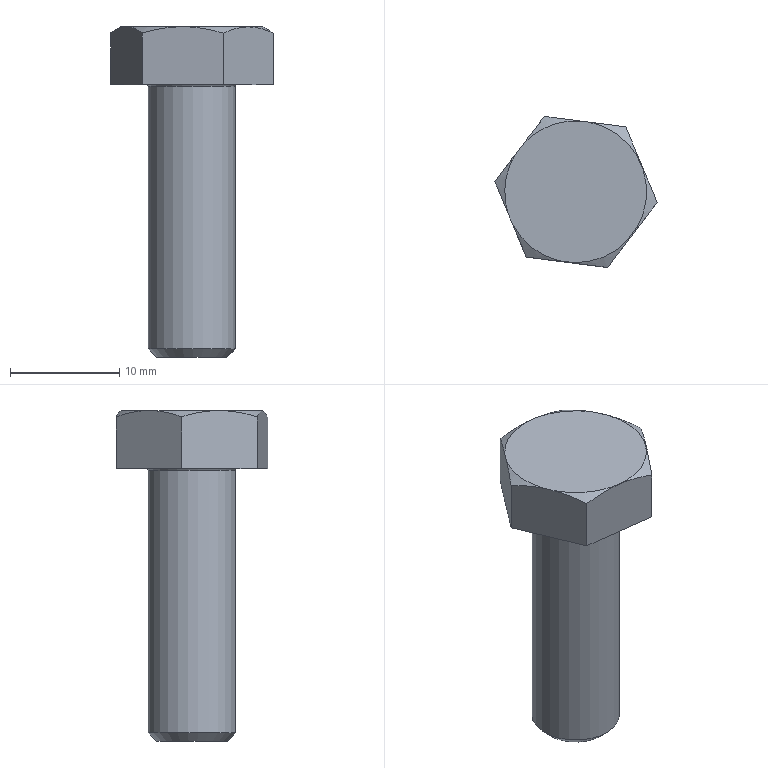Component | NX | 3_BOLT_3 | 1 solid | 15 faces | volume 2023 mm3 | plane 9 | other 3 | cylinder 1 | cone 1 | torus 1 | commonest cylinder face diameters 8 x1